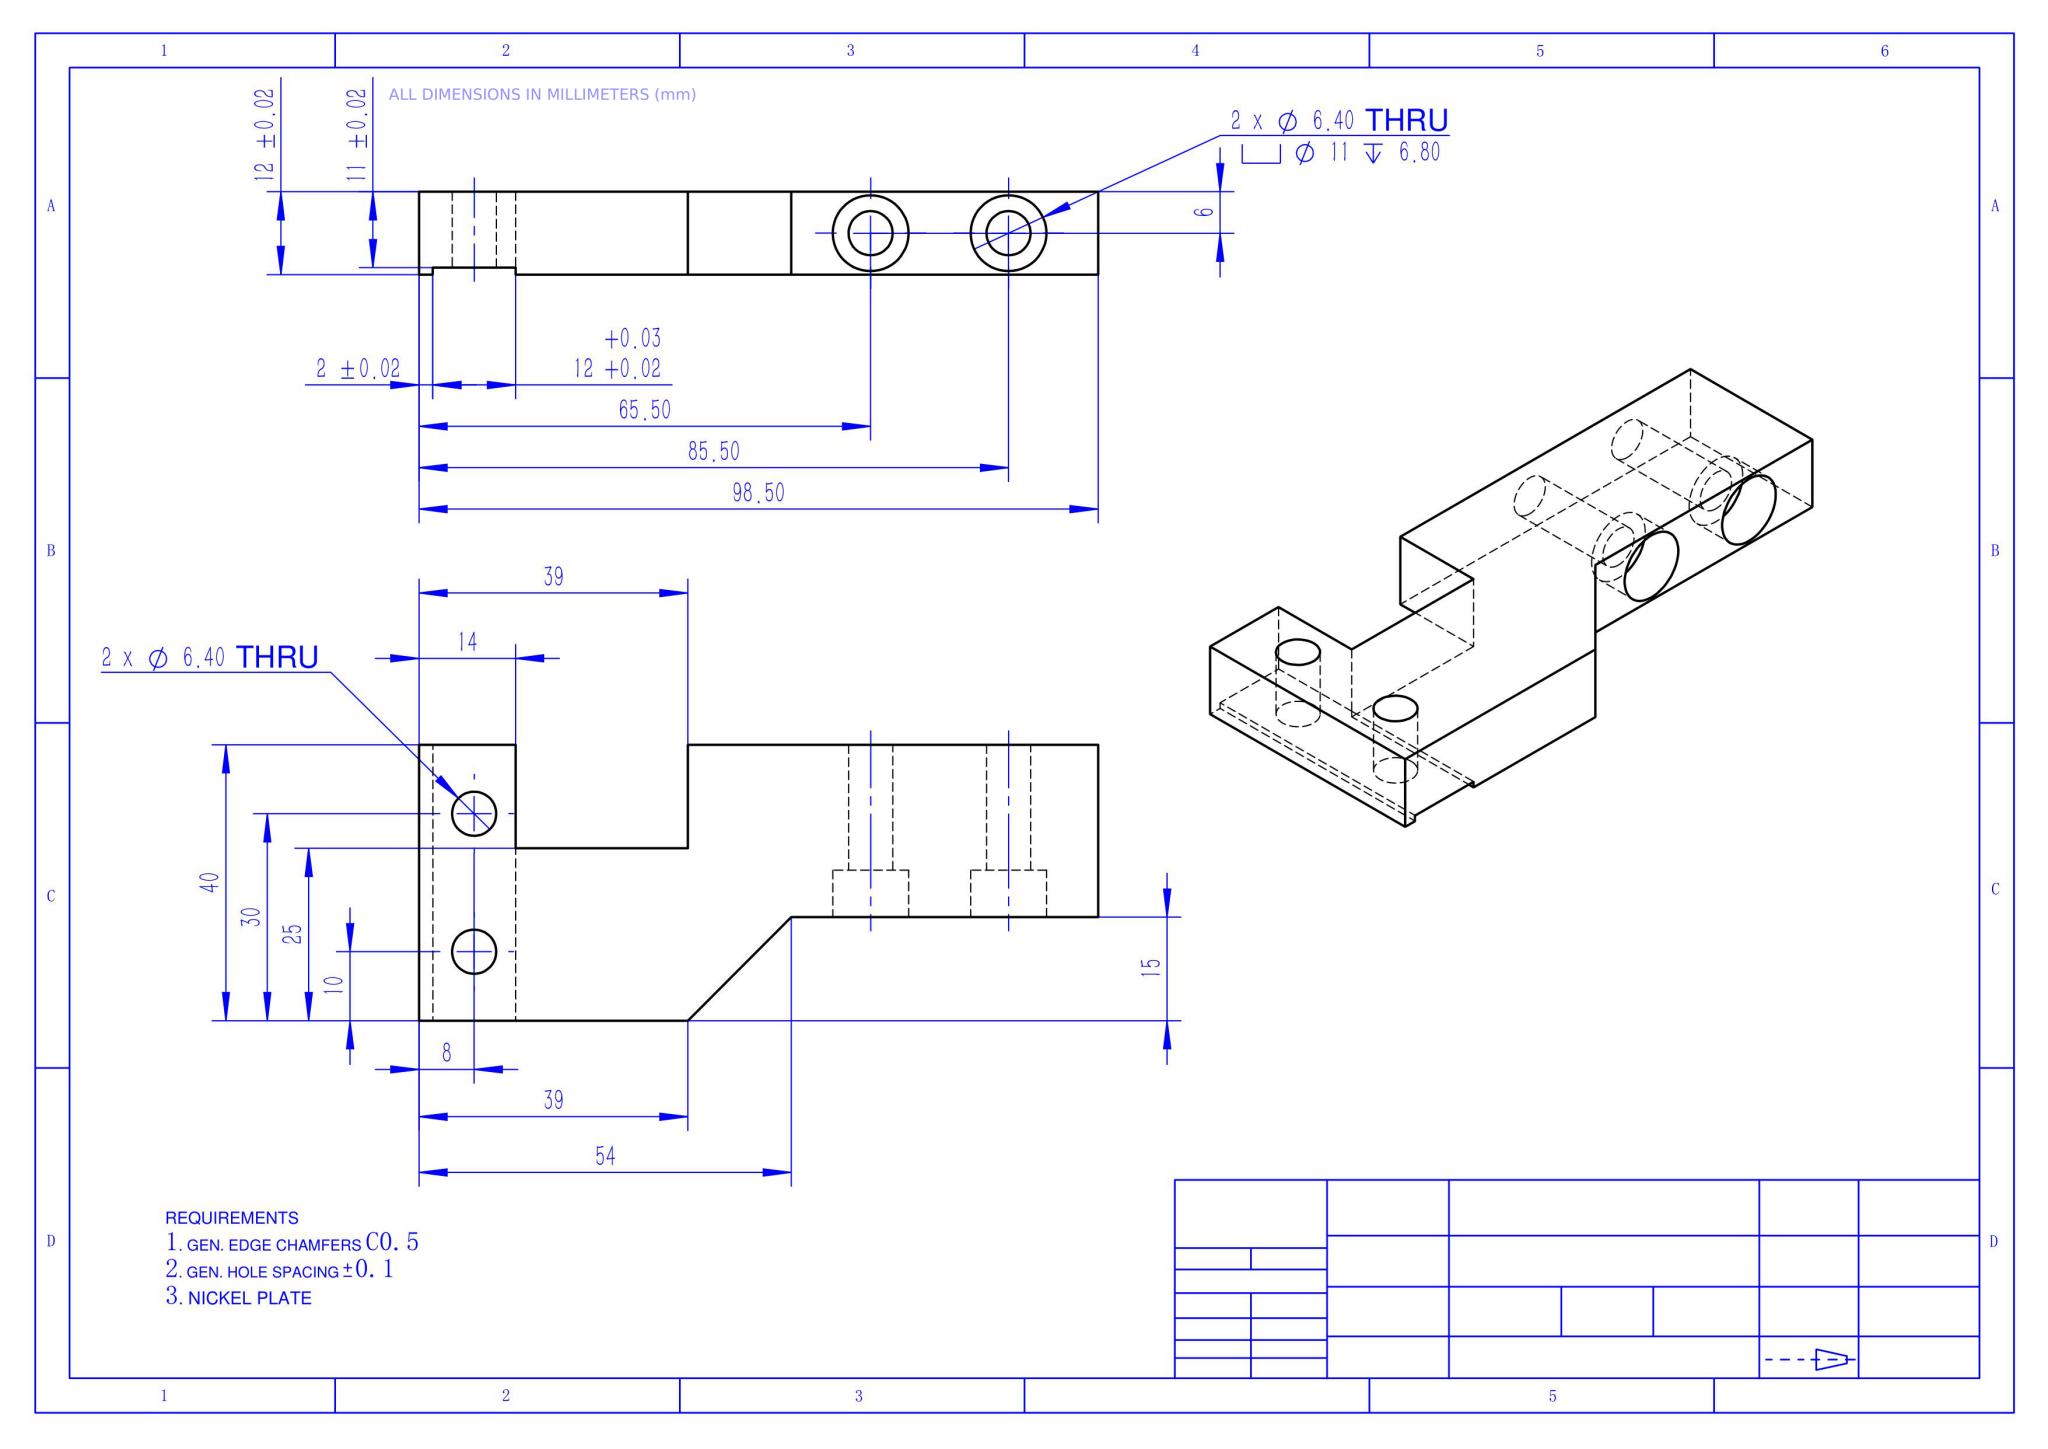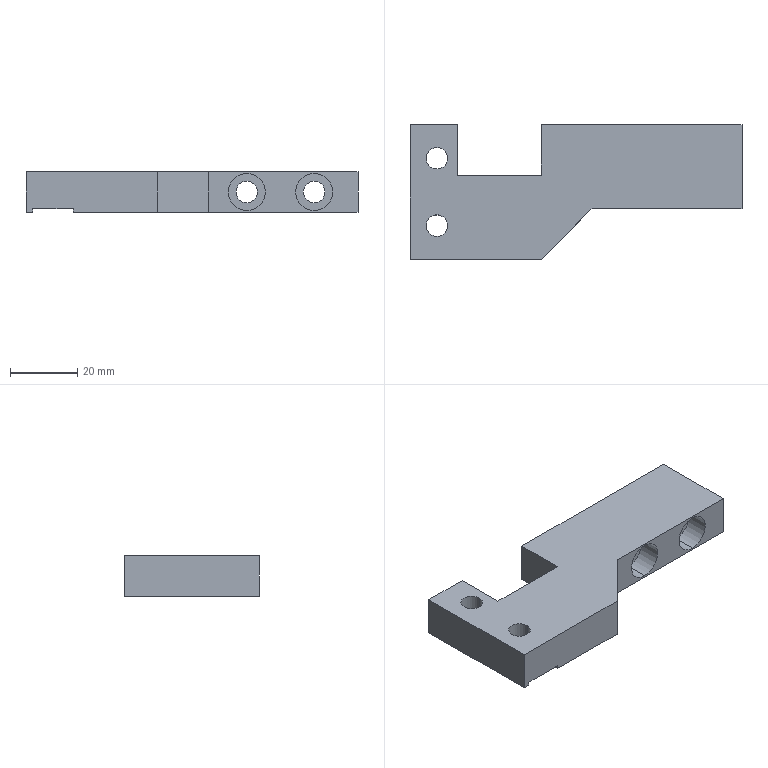Part | NX | mm | 1 solid | 30 faces | box 98.5 x 40 x 12 mm | volume 29769 mm3 | plane 18 | cylinder 12 | commonest cylinder face diameters 6.4 x8 11 x4
STEP:
#1=COLOUR_RGB('',0.698,0.698,0.698);
#2=FILL_AREA_STYLE_COLOUR('',#1);
#3=FILL_AREA_STYLE('',(#2));
#4=SURFACE_STYLE_FILL_AREA(#3);
#5=SURFACE_SIDE_STYLE('',(#4));
#6=SURFACE_STYLE_USAGE(.BOTH.,#5);
#7=PRESENTATION_STYLE_ASSIGNMENT((#6));
#8=CARTESIAN_POINT('',(85.5,1.8,11.5));
#9=VERTEX_POINT('',#8);
#10=CARTESIAN_POINT('',(85.5,1.8,0.5));
#11=VERTEX_POINT('',#10);
#12=CARTESIAN_POINT('',(85.5,1.8,6.));
#13=DIRECTION('',(0.,-1.,0.));
#14=DIRECTION('',(0.,0.,-1.));
#15=AXIS2_PLACEMENT_3D('',#12,#13,#14);
#16=CIRCLE('',#15,5.5);
#17=EDGE_CURVE('',#9,#11,#16,.T.);
#18=ORIENTED_EDGE('',*,*,#17,.F.);
#19=CARTESIAN_POINT('',(85.5,-5.,11.5));
#20=VERTEX_POINT('',#19);
#21=CARTESIAN_POINT('',(85.5,-5.,11.5));
#22=DIRECTION('',(0.,-1.,0.));
#23=VECTOR('',#22,1000.);
#24=LINE('',#21,#23);
#25=EDGE_CURVE('',#9,#20,#24,.T.);
#26=ORIENTED_EDGE('',*,*,#25,.T.);
#27=CARTESIAN_POINT('',(85.5,-5.,0.5));
#28=VERTEX_POINT('',#27);
#29=CARTESIAN_POINT('',(85.5,-5.,6.));
#30=DIRECTION('',(0.,-1.,0.));
#31=DIRECTION('',(0.,0.,-1.));
#32=AXIS2_PLACEMENT_3D('',#29,#30,#31);
#33=CIRCLE('',#32,5.5);
#34=EDGE_CURVE('',#20,#28,#33,.T.);
#35=ORIENTED_EDGE('',*,*,#34,.T.);
#36=CARTESIAN_POINT('',(85.5,-5.,0.5));
#37=DIRECTION('',(0.,-1.,0.));
#38=VECTOR('',#37,1000.);
#39=LINE('',#36,#38);
#40=EDGE_CURVE('',#11,#28,#39,.T.);
#41=ORIENTED_EDGE('',*,*,#40,.F.);
#42=EDGE_LOOP('',(#18,#26,#35,#41));
#43=FACE_OUTER_BOUND('',#42,.T.);
#44=CARTESIAN_POINT('',(85.5,-5.,6.));
#45=DIRECTION('',(0.,-1.,0.));
#46=DIRECTION('',(0.,0.,-1.));
#47=AXIS2_PLACEMENT_3D('',#44,#45,#46);
#48=CYLINDRICAL_SURFACE('',#47,5.5);
#49=ADVANCED_FACE('',(#43),#48,.F.);
#50=CARTESIAN_POINT('',(85.5,20.,9.2));
#51=VERTEX_POINT('',#50);
#52=CARTESIAN_POINT('',(85.5,20.,2.8));
#53=VERTEX_POINT('',#52);
#54=CARTESIAN_POINT('',(85.5,20.,6.));
#55=DIRECTION('',(0.,-1.,0.));
#56=DIRECTION('',(0.,0.,-1.));
#57=AXIS2_PLACEMENT_3D('',#54,#55,#56);
#58=CIRCLE('',#57,3.2);
#59=EDGE_CURVE('',#51,#53,#58,.T.);
#60=ORIENTED_EDGE('',*,*,#59,.F.);
#61=CARTESIAN_POINT('',(85.5,1.8,9.2));
#62=VERTEX_POINT('',#61);
#63=CARTESIAN_POINT('',(85.5,-5.,9.2));
#64=DIRECTION('',(0.,-1.,0.));
#65=VECTOR('',#64,1000.);
#66=LINE('',#63,#65);
#67=EDGE_CURVE('',#51,#62,#66,.T.);
#68=ORIENTED_EDGE('',*,*,#67,.T.);
#69=CARTESIAN_POINT('',(85.5,1.8,2.8));
#70=VERTEX_POINT('',#69);
#71=CARTESIAN_POINT('',(85.5,1.8,6.));
#72=DIRECTION('',(0.,-1.,0.));
#73=DIRECTION('',(0.,0.,-1.));
#74=AXIS2_PLACEMENT_3D('',#71,#72,#73);
#75=CIRCLE('',#74,3.2);
#76=EDGE_CURVE('',#62,#70,#75,.T.);
#77=ORIENTED_EDGE('',*,*,#76,.T.);
#78=CARTESIAN_POINT('',(85.5,-5.,2.8));
#79=DIRECTION('',(0.,-1.,0.));
#80=VECTOR('',#79,1000.);
#81=LINE('',#78,#80);
#82=EDGE_CURVE('',#53,#70,#81,.T.);
#83=ORIENTED_EDGE('',*,*,#82,.F.);
#84=EDGE_LOOP('',(#60,#68,#77,#83));
#85=FACE_OUTER_BOUND('',#84,.T.);
#86=CARTESIAN_POINT('',(85.5,-5.,6.));
#87=DIRECTION('',(0.,-1.,0.));
#88=DIRECTION('',(0.,0.,-1.));
#89=AXIS2_PLACEMENT_3D('',#86,#87,#88);
#90=CYLINDRICAL_SURFACE('',#89,3.2);
#91=ADVANCED_FACE('',(#85),#90,.F.);
#92=CARTESIAN_POINT('',(65.5,1.8,11.5));
#93=VERTEX_POINT('',#92);
#94=CARTESIAN_POINT('',(65.5,1.8,0.5));
#95=VERTEX_POINT('',#94);
#96=CARTESIAN_POINT('',(65.5,1.8,6.));
#97=DIRECTION('',(0.,-1.,0.));
#98=DIRECTION('',(0.,0.,-1.));
#99=AXIS2_PLACEMENT_3D('',#96,#97,#98);
#100=CIRCLE('',#99,5.5);
#101=EDGE_CURVE('',#93,#95,#100,.T.);
#102=ORIENTED_EDGE('',*,*,#101,.F.);
#103=CARTESIAN_POINT('',(65.5,-5.,11.5));
#104=VERTEX_POINT('',#103);
#105=CARTESIAN_POINT('',(65.5,-5.,11.5));
#106=DIRECTION('',(0.,-1.,0.));
#107=VECTOR('',#106,1000.);
#108=LINE('',#105,#107);
#109=EDGE_CURVE('',#93,#104,#108,.T.);
#110=ORIENTED_EDGE('',*,*,#109,.T.);
#111=CARTESIAN_POINT('',(65.5,-5.,0.5));
#112=VERTEX_POINT('',#111);
#113=CARTESIAN_POINT('',(65.5,-5.,6.));
#114=DIRECTION('',(0.,-1.,0.));
#115=DIRECTION('',(0.,0.,-1.));
#116=AXIS2_PLACEMENT_3D('',#113,#114,#115);
#117=CIRCLE('',#116,5.5);
#118=EDGE_CURVE('',#104,#112,#117,.T.);
#119=ORIENTED_EDGE('',*,*,#118,.T.);
#120=CARTESIAN_POINT('',(65.5,-5.,0.5));
#121=DIRECTION('',(0.,-1.,0.));
#122=VECTOR('',#121,1000.);
#123=LINE('',#120,#122);
#124=EDGE_CURVE('',#95,#112,#123,.T.);
#125=ORIENTED_EDGE('',*,*,#124,.F.);
#126=EDGE_LOOP('',(#102,#110,#119,#125));
#127=FACE_OUTER_BOUND('',#126,.T.);
#128=CARTESIAN_POINT('',(65.5,-5.,6.));
#129=DIRECTION('',(0.,-1.,0.));
#130=DIRECTION('',(0.,0.,-1.));
#131=AXIS2_PLACEMENT_3D('',#128,#129,#130);
#132=CYLINDRICAL_SURFACE('',#131,5.5);
#133=ADVANCED_FACE('',(#127),#132,.F.);
#134=CARTESIAN_POINT('',(65.5,20.,9.2));
#135=VERTEX_POINT('',#134);
#136=CARTESIAN_POINT('',(65.5,20.,2.8));
#137=VERTEX_POINT('',#136);
#138=CARTESIAN_POINT('',(65.5,20.,6.));
#139=DIRECTION('',(0.,-1.,0.));
#140=DIRECTION('',(0.,0.,-1.));
#141=AXIS2_PLACEMENT_3D('',#138,#139,#140);
#142=CIRCLE('',#141,3.2);
#143=EDGE_CURVE('',#135,#137,#142,.T.);
#144=ORIENTED_EDGE('',*,*,#143,.F.);
#145=CARTESIAN_POINT('',(65.5,1.8,9.2));
#146=VERTEX_POINT('',#145);
#147=CARTESIAN_POINT('',(65.5,-5.,9.2));
#148=DIRECTION('',(0.,-1.,0.));
#149=VECTOR('',#148,1000.);
#150=LINE('',#147,#149);
#151=EDGE_CURVE('',#135,#146,#150,.T.);
#152=ORIENTED_EDGE('',*,*,#151,.T.);
#153=CARTESIAN_POINT('',(65.5,1.8,2.8));
#154=VERTEX_POINT('',#153);
#155=CARTESIAN_POINT('',(65.5,1.8,6.));
#156=DIRECTION('',(0.,-1.,0.));
#157=DIRECTION('',(0.,0.,-1.));
#158=AXIS2_PLACEMENT_3D('',#155,#156,#157);
#159=CIRCLE('',#158,3.2);
#160=EDGE_CURVE('',#146,#154,#159,.T.);
#161=ORIENTED_EDGE('',*,*,#160,.T.);
#162=CARTESIAN_POINT('',(65.5,-5.,2.8));
#163=DIRECTION('',(0.,-1.,0.));
#164=VECTOR('',#163,1000.);
#165=LINE('',#162,#164);
#166=EDGE_CURVE('',#137,#154,#165,.T.);
#167=ORIENTED_EDGE('',*,*,#166,.F.);
#168=EDGE_LOOP('',(#144,#152,#161,#167));
#169=FACE_OUTER_BOUND('',#168,.T.);
#170=CARTESIAN_POINT('',(65.5,-5.,6.));
#171=DIRECTION('',(0.,-1.,0.));
#172=DIRECTION('',(0.,0.,-1.));
#173=AXIS2_PLACEMENT_3D('',#170,#171,#172);
#174=CYLINDRICAL_SURFACE('',#173,3.2);
#175=ADVANCED_FACE('',(#169),#174,.F.);
#176=CARTESIAN_POINT('',(4.8,10.,1.));
#177=VERTEX_POINT('',#176);
#178=CARTESIAN_POINT('',(11.2,10.,1.));
#179=VERTEX_POINT('',#178);
#180=CARTESIAN_POINT('',(8.,10.,1.));
#181=DIRECTION('',(0.,0.,1.));
#182=DIRECTION('',(1.,0.,0.));
#183=AXIS2_PLACEMENT_3D('',#180,#181,#182);
#184=CIRCLE('',#183,3.2);
#185=EDGE_CURVE('',#177,#179,#184,.T.);
#186=ORIENTED_EDGE('',*,*,#185,.F.);
#187=CARTESIAN_POINT('',(4.8,10.,12.));
#188=VERTEX_POINT('',#187);
#189=CARTESIAN_POINT('',(4.8,10.,12.));
#190=DIRECTION('',(0.,0.,1.));
#191=VECTOR('',#190,1000.);
#192=LINE('',#189,#191);
#193=EDGE_CURVE('',#177,#188,#192,.T.);
#194=ORIENTED_EDGE('',*,*,#193,.T.);
#195=CARTESIAN_POINT('',(11.2,10.,12.));
#196=VERTEX_POINT('',#195);
#197=CARTESIAN_POINT('',(8.,10.,12.));
#198=DIRECTION('',(0.,0.,1.));
#199=DIRECTION('',(1.,0.,0.));
#200=AXIS2_PLACEMENT_3D('',#197,#198,#199);
#201=CIRCLE('',#200,3.2);
#202=EDGE_CURVE('',#188,#196,#201,.T.);
#203=ORIENTED_EDGE('',*,*,#202,.T.);
#204=CARTESIAN_POINT('',(11.2,10.,12.));
#205=DIRECTION('',(0.,0.,1.));
#206=VECTOR('',#205,1000.);
#207=LINE('',#204,#206);
#208=EDGE_CURVE('',#179,#196,#207,.T.);
#209=ORIENTED_EDGE('',*,*,#208,.F.);
#210=EDGE_LOOP('',(#186,#194,#203,#209));
#211=FACE_OUTER_BOUND('',#210,.T.);
#212=CARTESIAN_POINT('',(8.,10.,12.));
#213=DIRECTION('',(0.,0.,1.));
#214=DIRECTION('',(1.,0.,0.));
#215=AXIS2_PLACEMENT_3D('',#212,#213,#214);
#216=CYLINDRICAL_SURFACE('',#215,3.2);
#217=ADVANCED_FACE('',(#211),#216,.F.);
#218=CARTESIAN_POINT('',(4.8,-10.,1.));
#219=VERTEX_POINT('',#218);
#220=CARTESIAN_POINT('',(11.2,-10.,1.));
#221=VERTEX_POINT('',#220);
#222=CARTESIAN_POINT('',(8.,-10.,1.));
#223=DIRECTION('',(0.,0.,1.));
#224=DIRECTION('',(1.,0.,0.));
#225=AXIS2_PLACEMENT_3D('',#222,#223,#224);
#226=CIRCLE('',#225,3.2);
#227=EDGE_CURVE('',#219,#221,#226,.T.);
#228=ORIENTED_EDGE('',*,*,#227,.F.);
#229=CARTESIAN_POINT('',(4.8,-10.,12.));
#230=VERTEX_POINT('',#229);
#231=CARTESIAN_POINT('',(4.8,-10.,12.));
#232=DIRECTION('',(0.,0.,1.));
#233=VECTOR('',#232,1000.);
#234=LINE('',#231,#233);
#235=EDGE_CURVE('',#219,#230,#234,.T.);
#236=ORIENTED_EDGE('',*,*,#235,.T.);
#237=CARTESIAN_POINT('',(11.2,-10.,12.));
#238=VERTEX_POINT('',#237);
#239=CARTESIAN_POINT('',(8.,-10.,12.));
#240=DIRECTION('',(0.,0.,1.));
#241=DIRECTION('',(1.,0.,0.));
#242=AXIS2_PLACEMENT_3D('',#239,#240,#241);
#243=CIRCLE('',#242,3.2);
#244=EDGE_CURVE('',#230,#238,#243,.T.);
#245=ORIENTED_EDGE('',*,*,#244,.T.);
#246=CARTESIAN_POINT('',(11.2,-10.,12.));
#247=DIRECTION('',(0.,0.,1.));
#248=VECTOR('',#247,1000.);
#249=LINE('',#246,#248);
#250=EDGE_CURVE('',#221,#238,#249,.T.);
#251=ORIENTED_EDGE('',*,*,#250,.F.);
#252=EDGE_LOOP('',(#228,#236,#245,#251));
#253=FACE_OUTER_BOUND('',#252,.T.);
#254=CARTESIAN_POINT('',(8.,-10.,12.));
#255=DIRECTION('',(0.,0.,1.));
#256=DIRECTION('',(1.,0.,0.));
#257=AXIS2_PLACEMENT_3D('',#254,#255,#256);
#258=CYLINDRICAL_SURFACE('',#257,3.2);
#259=ADVANCED_FACE('',(#253),#258,.F.);
#260=CARTESIAN_POINT('',(14.,20.,12.));
#261=VERTEX_POINT('',#260);
#262=CARTESIAN_POINT('',(0.,20.,12.));
#263=VERTEX_POINT('',#262);
#264=CARTESIAN_POINT('',(0.,20.,12.));
#265=DIRECTION('',(-1.,0.,0.));
#266=VECTOR('',#265,1000.);
#267=LINE('',#264,#266);
#268=EDGE_CURVE('',#261,#263,#267,.T.);
#269=ORIENTED_EDGE('',*,*,#268,.F.);
#270=CARTESIAN_POINT('',(14.,20.,1.));
#271=VERTEX_POINT('',#270);
#272=CARTESIAN_POINT('',(14.,20.,12.));
#273=DIRECTION('',(0.,0.,-1.));
#274=VECTOR('',#273,1000.);
#275=LINE('',#272,#274);
#276=EDGE_CURVE('',#261,#271,#275,.T.);
#277=ORIENTED_EDGE('',*,*,#276,.T.);
#278=CARTESIAN_POINT('',(2.,20.,1.));
#279=VERTEX_POINT('',#278);
#280=CARTESIAN_POINT('',(2.,20.,1.));
#281=DIRECTION('',(1.,0.,0.));
#282=VECTOR('',#281,1000.);
#283=LINE('',#280,#282);
#284=EDGE_CURVE('',#279,#271,#283,.T.);
#285=ORIENTED_EDGE('',*,*,#284,.F.);
#286=CARTESIAN_POINT('',(2.,20.,0.));
#287=VERTEX_POINT('',#286);
#288=CARTESIAN_POINT('',(2.,20.,1.));
#289=DIRECTION('',(0.,0.,-1.));
#290=VECTOR('',#289,1000.);
#291=LINE('',#288,#290);
#292=EDGE_CURVE('',#279,#287,#291,.T.);
#293=ORIENTED_EDGE('',*,*,#292,.T.);
#294=CARTESIAN_POINT('',(0.,20.,0.));
#295=VERTEX_POINT('',#294);
#296=CARTESIAN_POINT('',(0.,20.,0.));
#297=DIRECTION('',(-1.,0.,0.));
#298=VECTOR('',#297,1000.);
#299=LINE('',#296,#298);
#300=EDGE_CURVE('',#287,#295,#299,.T.);
#301=ORIENTED_EDGE('',*,*,#300,.T.);
#302=CARTESIAN_POINT('',(0.,20.,12.));
#303=DIRECTION('',(0.,0.,-1.));
#304=VECTOR('',#303,1000.);
#305=LINE('',#302,#304);
#306=EDGE_CURVE('',#263,#295,#305,.T.);
#307=ORIENTED_EDGE('',*,*,#306,.F.);
#308=EDGE_LOOP('',(#269,#277,#285,#293,#301,#307));
#309=FACE_OUTER_BOUND('',#308,.T.);
#310=CARTESIAN_POINT('',(0.,20.,12.));
#311=DIRECTION('',(0.,-1.,0.));
#312=DIRECTION('',(0.,0.,-1.));
#313=AXIS2_PLACEMENT_3D('',#310,#311,#312);
#314=PLANE('',#313);
#315=ADVANCED_FACE('',(#309),#314,.F.);
#316=ORIENTED_EDGE('',*,*,#300,.F.);
#317=CARTESIAN_POINT('',(2.,-20.,0.));
#318=VERTEX_POINT('',#317);
#319=CARTESIAN_POINT('',(2.,20.,0.));
#320=DIRECTION('',(0.,1.,0.));
#321=VECTOR('',#320,1000.);
#322=LINE('',#319,#321);
#323=EDGE_CURVE('',#318,#287,#322,.T.);
#324=ORIENTED_EDGE('',*,*,#323,.F.);
#325=CARTESIAN_POINT('',(0.,-20.,0.));
#326=VERTEX_POINT('',#325);
#327=CARTESIAN_POINT('',(0.,-20.,0.));
#328=DIRECTION('',(1.,0.,0.));
#329=VECTOR('',#328,1000.);
#330=LINE('',#327,#329);
#331=EDGE_CURVE('',#326,#318,#330,.T.);
#332=ORIENTED_EDGE('',*,*,#331,.F.);
#333=CARTESIAN_POINT('',(0.,20.,0.));
#334=DIRECTION('',(0.,-1.,0.));
#335=VECTOR('',#334,1000.);
#336=LINE('',#333,#335);
#337=EDGE_CURVE('',#295,#326,#336,.T.);
#338=ORIENTED_EDGE('',*,*,#337,.F.);
#339=EDGE_LOOP('',(#316,#324,#332,#338));
#340=FACE_OUTER_BOUND('',#339,.T.);
#341=CARTESIAN_POINT('',(0.,0.,0.));
#342=DIRECTION('',(0.,0.,1.));
#343=DIRECTION('',(1.,0.,0.));
#344=AXIS2_PLACEMENT_3D('',#341,#342,#343);
#345=PLANE('',#344);
#346=ADVANCED_FACE('',(#340),#345,.F.);
#347=ORIENTED_EDGE('',*,*,#337,.T.);
#348=CARTESIAN_POINT('',(0.,-20.,12.));
#349=VERTEX_POINT('',#348);
#350=CARTESIAN_POINT('',(0.,-20.,12.));
#351=DIRECTION('',(0.,0.,-1.));
#352=VECTOR('',#351,1000.);
#353=LINE('',#350,#352);
#354=EDGE_CURVE('',#349,#326,#353,.T.);
#355=ORIENTED_EDGE('',*,*,#354,.F.);
#356=CARTESIAN_POINT('',(0.,20.,12.));
#357=DIRECTION('',(0.,-1.,0.));
#358=VECTOR('',#357,1000.);
#359=LINE('',#356,#358);
#360=EDGE_CURVE('',#263,#349,#359,.T.);
#361=ORIENTED_EDGE('',*,*,#360,.F.);
#362=ORIENTED_EDGE('',*,*,#306,.T.);
#363=EDGE_LOOP('',(#347,#355,#361,#362));
#364=FACE_OUTER_BOUND('',#363,.T.);
#365=CARTESIAN_POINT('',(0.,20.,12.));
#366=DIRECTION('',(1.,0.,0.));
#367=DIRECTION('',(0.,0.,-1.));
#368=AXIS2_PLACEMENT_3D('',#365,#366,#367);
#369=PLANE('',#368);
#370=ADVANCED_FACE('',(#364),#369,.F.);
#371=CARTESIAN_POINT('',(14.,-20.,0.));
#372=VERTEX_POINT('',#371);
#373=CARTESIAN_POINT('',(39.,-20.,0.));
#374=VERTEX_POINT('',#373);
#375=CARTESIAN_POINT('',(0.,-20.,0.));
#376=DIRECTION('',(1.,0.,0.));
#377=VECTOR('',#376,1000.);
#378=LINE('',#375,#377);
#379=EDGE_CURVE('',#372,#374,#378,.T.);
#380=ORIENTED_EDGE('',*,*,#379,.T.);
#381=CARTESIAN_POINT('',(39.,-20.,12.));
#382=VERTEX_POINT('',#381);
#383=CARTESIAN_POINT('',(39.,-20.,12.));
#384=DIRECTION('',(0.,0.,1.));
#385=VECTOR('',#384,1000.);
#386=LINE('',#383,#385);
#387=EDGE_CURVE('',#374,#382,#386,.T.);
#388=ORIENTED_EDGE('',*,*,#387,.T.);
#389=CARTESIAN_POINT('',(0.,-20.,12.));
#390=DIRECTION('',(1.,0.,0.));
#391=VECTOR('',#390,1000.);
#392=LINE('',#389,#391);
#393=EDGE_CURVE('',#349,#382,#392,.T.);
#394=ORIENTED_EDGE('',*,*,#393,.F.);
#395=ORIENTED_EDGE('',*,*,#354,.T.);
#396=ORIENTED_EDGE('',*,*,#331,.T.);
#397=CARTESIAN_POINT('',(2.,-20.,1.));
#398=VERTEX_POINT('',#397);
#399=CARTESIAN_POINT('',(2.,-20.,1.));
#400=DIRECTION('',(0.,0.,-1.));
#401=VECTOR('',#400,1000.);
#402=LINE('',#399,#401);
#403=EDGE_CURVE('',#398,#318,#402,.T.);
#404=ORIENTED_EDGE('',*,*,#403,.F.);
#405=CARTESIAN_POINT('',(14.,-20.,1.));
#406=VERTEX_POINT('',#405);
#407=CARTESIAN_POINT('',(2.,-20.,1.));
#408=DIRECTION('',(-1.,0.,0.));
#409=VECTOR('',#408,1000.);
#410=LINE('',#407,#409);
#411=EDGE_CURVE('',#406,#398,#410,.T.);
#412=ORIENTED_EDGE('',*,*,#411,.F.);
#413=CARTESIAN_POINT('',(14.,-20.,1.));
#414=DIRECTION('',(0.,0.,-1.));
#415=VECTOR('',#414,1000.);
#416=LINE('',#413,#415);
#417=EDGE_CURVE('',#406,#372,#416,.T.);
#418=ORIENTED_EDGE('',*,*,#417,.T.);
#419=EDGE_LOOP('',(#380,#388,#394,#395,#396,#404,#412,#418));
#420=FACE_OUTER_BOUND('',#419,.T.);
#421=CARTESIAN_POINT('',(0.,-20.,12.));
#422=DIRECTION('',(0.,1.,0.));
#423=DIRECTION('',(0.,0.,1.));
#424=AXIS2_PLACEMENT_3D('',#421,#422,#423);
#425=PLANE('',#424);
#426=ADVANCED_FACE('',(#420),#425,.F.);
#427=CARTESIAN_POINT('',(98.5,-5.,12.));
#428=VERTEX_POINT('',#427);
#429=CARTESIAN_POINT('',(98.5,20.,12.));
#430=VERTEX_POINT('',#429);
#431=CARTESIAN_POINT('',(98.5,20.,12.));
#432=DIRECTION('',(0.,1.,0.));
#433=VECTOR('',#432,1000.);
#434=LINE('',#431,#433);
#435=EDGE_CURVE('',#428,#430,#434,.T.);
#436=ORIENTED_EDGE('',*,*,#435,.F.);
#437=CARTESIAN_POINT('',(98.5,-5.,0.));
#438=VERTEX_POINT('',#437);
#439=CARTESIAN_POINT('',(98.5,-5.,0.));
#440=DIRECTION('',(0.,0.,1.));
#441=VECTOR('',#440,1000.);
#442=LINE('',#439,#441);
#443=EDGE_CURVE('',#438,#428,#442,.T.);
#444=ORIENTED_EDGE('',*,*,#443,.F.);
#445=CARTESIAN_POINT('',(98.5,20.,0.));
#446=VERTEX_POINT('',#445);
#447=CARTESIAN_POINT('',(98.5,20.,0.));
#448=DIRECTION('',(0.,1.,0.));
#449=VECTOR('',#448,1000.);
#450=LINE('',#447,#449);
#451=EDGE_CURVE('',#438,#446,#450,.T.);
#452=ORIENTED_EDGE('',*,*,#451,.T.);
#453=CARTESIAN_POINT('',(98.5,20.,12.));
#454=DIRECTION('',(0.,0.,-1.));
#455=VECTOR('',#454,1000.);
#456=LINE('',#453,#455);
#457=EDGE_CURVE('',#430,#446,#456,.T.);
#458=ORIENTED_EDGE('',*,*,#457,.F.);
#459=EDGE_LOOP('',(#436,#444,#452,#458));
#460=FACE_OUTER_BOUND('',#459,.T.);
#461=CARTESIAN_POINT('',(98.5,20.,12.));
#462=DIRECTION('',(-1.,0.,0.));
#463=DIRECTION('',(0.,0.,1.));
#464=AXIS2_PLACEMENT_3D('',#461,#462,#463);
#465=PLANE('',#464);
#466=ADVANCED_FACE('',(#460),#465,.F.);
#467=CARTESIAN_POINT('',(85.5,20.,6.));
#468=DIRECTION('',(0.,-1.,0.));
#469=DIRECTION('',(0.,0.,-1.));
#470=AXIS2_PLACEMENT_3D('',#467,#468,#469);
#471=CIRCLE('',#470,3.2);
#472=EDGE_CURVE('',#53,#51,#471,.T.);
#473=ORIENTED_EDGE('',*,*,#472,.T.);
#474=ORIENTED_EDGE('',*,*,#59,.T.);
#475=EDGE_LOOP('',(#473,#474));
#476=FACE_BOUND('',#475,.T.);
#477=CARTESIAN_POINT('',(65.5,20.,6.));
#478=DIRECTION('',(0.,-1.,0.));
#479=DIRECTION('',(0.,0.,-1.));
#480=AXIS2_PLACEMENT_3D('',#477,#478,#479);
#481=CIRCLE('',#480,3.2);
#482=EDGE_CURVE('',#137,#135,#481,.T.);
#483=ORIENTED_EDGE('',*,*,#482,.T.);
#484=ORIENTED_EDGE('',*,*,#143,.T.);
#485=EDGE_LOOP('',(#483,#484));
#486=FACE_BOUND('',#485,.T.);
#487=CARTESIAN_POINT('',(39.,20.,0.));
#488=VERTEX_POINT('',#487);
#489=CARTESIAN_POINT('',(0.,20.,0.));
#490=DIRECTION('',(-1.,0.,0.));
#491=VECTOR('',#490,1000.);
#492=LINE('',#489,#491);
#493=EDGE_CURVE('',#446,#488,#492,.T.);
#494=ORIENTED_EDGE('',*,*,#493,.T.);
#495=CARTESIAN_POINT('',(39.,20.,12.));
#496=VERTEX_POINT('',#495);
#497=CARTESIAN_POINT('',(39.,20.,12.));
#498=DIRECTION('',(0.,0.,-1.));
#499=VECTOR('',#498,1000.);
#500=LINE('',#497,#499);
#501=EDGE_CURVE('',#496,#488,#500,.T.);
#502=ORIENTED_EDGE('',*,*,#501,.F.);
#503=CARTESIAN_POINT('',(0.,20.,12.));
#504=DIRECTION('',(-1.,0.,0.));
#505=VECTOR('',#504,1000.);
#506=LINE('',#503,#505);
#507=EDGE_CURVE('',#430,#496,#506,.T.);
#508=ORIENTED_EDGE('',*,*,#507,.F.);
#509=ORIENTED_EDGE('',*,*,#457,.T.);
#510=EDGE_LOOP('',(#494,#502,#508,#509));
#511=FACE_OUTER_BOUND('',#510,.T.);
#512=CARTESIAN_POINT('',(0.,20.,12.));
#513=DIRECTION('',(0.,-1.,0.));
#514=DIRECTION('',(0.,0.,-1.));
#515=AXIS2_PLACEMENT_3D('',#512,#513,#514);
#516=PLANE('',#515);
#517=ADVANCED_FACE('',(#476,#486,#511),#516,.F.);
#518=ORIENTED_EDGE('',*,*,#393,.T.);
#519=CARTESIAN_POINT('',(54.,-5.,12.));
#520=VERTEX_POINT('',#519);
#521=CARTESIAN_POINT('',(29.5,-29.5,12.));
#522=DIRECTION('',(0.7071,0.7071,0.));
#523=VECTOR('',#522,1000.);
#524=LINE('',#521,#523);
#525=EDGE_CURVE('',#382,#520,#524,.T.);
#526=ORIENTED_EDGE('',*,*,#525,.T.);
#527=CARTESIAN_POINT('',(98.5,-5.,12.));
#528=DIRECTION('',(-1.,-0.,0.));
#529=VECTOR('',#528,1000.);
#530=LINE('',#527,#529);
#531=EDGE_CURVE('',#428,#520,#530,.T.);
#532=ORIENTED_EDGE('',*,*,#531,.F.);
#533=ORIENTED_EDGE('',*,*,#435,.T.);
#534=ORIENTED_EDGE('',*,*,#507,.T.);
#535=CARTESIAN_POINT('',(39.,5.,12.));
#536=VERTEX_POINT('',#535);
#537=CARTESIAN_POINT('',(39.,20.,12.));
#538=DIRECTION('',(0.,-1.,0.));
#539=VECTOR('',#538,1000.);
#540=LINE('',#537,#539);
#541=EDGE_CURVE('',#496,#536,#540,.T.);
#542=ORIENTED_EDGE('',*,*,#541,.T.);
#543=CARTESIAN_POINT('',(14.,5.,12.));
#544=VERTEX_POINT('',#543);
#545=CARTESIAN_POINT('',(14.,5.,12.));
#546=DIRECTION('',(-1.,-0.,0.));
#547=VECTOR('',#546,1000.);
#548=LINE('',#545,#547);
#549=EDGE_CURVE('',#536,#544,#548,.T.);
#550=ORIENTED_EDGE('',*,*,#549,.T.);
#551=CARTESIAN_POINT('',(14.,20.,12.));
#552=DIRECTION('',(0.,1.,0.));
#553=VECTOR('',#552,1000.);
#554=LINE('',#551,#553);
#555=EDGE_CURVE('',#544,#261,#554,.T.);
#556=ORIENTED_EDGE('',*,*,#555,.T.);
#557=ORIENTED_EDGE('',*,*,#268,.T.);
#558=ORIENTED_EDGE('',*,*,#360,.T.);
#559=EDGE_LOOP('',(#518,#526,#532,#533,#534,#542,#550,#556,#557,#558));
#560=FACE_OUTER_BOUND('',#559,.T.);
#561=CARTESIAN_POINT('',(8.,10.,12.));
#562=DIRECTION('',(0.,0.,1.));
#563=DIRECTION('',(1.,0.,0.));
#564=AXIS2_PLACEMENT_3D('',#561,#562,#563);
#565=CIRCLE('',#564,3.2);
#566=EDGE_CURVE('',#196,#188,#565,.T.);
#567=ORIENTED_EDGE('',*,*,#566,.F.);
#568=ORIENTED_EDGE('',*,*,#202,.F.);
#569=EDGE_LOOP('',(#567,#568));
#570=FACE_BOUND('',#569,.T.);
#571=CARTESIAN_POINT('',(8.,-10.,12.));
#572=DIRECTION('',(0.,0.,1.));
#573=DIRECTION('',(1.,0.,0.));
#574=AXIS2_PLACEMENT_3D('',#571,#572,#573);
#575=CIRCLE('',#574,3.2);
#576=EDGE_CURVE('',#238,#230,#575,.T.);
#577=ORIENTED_EDGE('',*,*,#576,.F.);
#578=ORIENTED_EDGE('',*,*,#244,.F.);
#579=EDGE_LOOP('',(#577,#578));
#580=FACE_BOUND('',#579,.T.);
#581=CARTESIAN_POINT('',(0.,0.,12.));
#582=DIRECTION('',(0.,0.,1.));
#583=DIRECTION('',(1.,0.,0.));
#584=AXIS2_PLACEMENT_3D('',#581,#582,#583);
#585=PLANE('',#584);
#586=ADVANCED_FACE('',(#560,#570,#580),#585,.T.);
#587=CARTESIAN_POINT('',(54.,-5.,0.));
#588=VERTEX_POINT('',#587);
#589=CARTESIAN_POINT('',(98.5,-5.,0.));
#590=DIRECTION('',(-1.,-0.,0.));
#591=VECTOR('',#590,1000.);
#592=LINE('',#589,#591);
#593=EDGE_CURVE('',#438,#588,#592,.T.);
#594=ORIENTED_EDGE('',*,*,#593,.T.);
#595=CARTESIAN_POINT('',(39.,-20.,0.));
#596=DIRECTION('',(-0.7071,-0.7071,0.));
#597=VECTOR('',#596,1000.);
#598=LINE('',#595,#597);
#599=EDGE_CURVE('',#588,#374,#598,.T.);
#600=ORIENTED_EDGE('',*,*,#599,.T.);
#601=ORIENTED_EDGE('',*,*,#379,.F.);
#602=CARTESIAN_POINT('',(14.,5.,0.));
#603=VERTEX_POINT('',#602);
#604=CARTESIAN_POINT('',(14.,20.,0.));
#605=DIRECTION('',(-0.,-1.,0.));
#606=VECTOR('',#605,1000.);
#607=LINE('',#604,#606);
#608=EDGE_CURVE('',#603,#372,#607,.T.);
#609=ORIENTED_EDGE('',*,*,#608,.F.);
#610=CARTESIAN_POINT('',(39.,5.,0.));
#611=VERTEX_POINT('',#610);
#612=CARTESIAN_POINT('',(14.,5.,0.));
#613=DIRECTION('',(-1.,-0.,0.));
#614=VECTOR('',#613,1000.);
#615=LINE('',#612,#614);
#616=EDGE_CURVE('',#611,#603,#615,.T.);
#617=ORIENTED_EDGE('',*,*,#616,.F.);
#618=CARTESIAN_POINT('',(39.,20.,0.));
#619=DIRECTION('',(0.,-1.,0.));
#620=VECTOR('',#619,1000.);
#621=LINE('',#618,#620);
#622=EDGE_CURVE('',#488,#611,#621,.T.);
#623=ORIENTED_EDGE('',*,*,#622,.F.);
#624=ORIENTED_EDGE('',*,*,#493,.F.);
#625=ORIENTED_EDGE('',*,*,#451,.F.);
#626=EDGE_LOOP('',(#594,#600,#601,#609,#617,#623,#624,#625));
#627=FACE_OUTER_BOUND('',#626,.T.);
#628=CARTESIAN_POINT('',(0.,0.,0.));
#629=DIRECTION('',(0.,0.,1.));
#630=DIRECTION('',(1.,0.,0.));
#631=AXIS2_PLACEMENT_3D('',#628,#629,#630);
#632=PLANE('',#631);
#633=ADVANCED_FACE('',(#627),#632,.F.);
#634=ORIENTED_EDGE('',*,*,#323,.T.);
#635=ORIENTED_EDGE('',*,*,#292,.F.);
#636=CARTESIAN_POINT('',(2.,20.,1.));
#637=DIRECTION('',(0.,1.,0.));
#638=VECTOR('',#637,1000.);
#639=LINE('',#636,#638);
#640=EDGE_CURVE('',#398,#279,#639,.T.);
#641=ORIENTED_EDGE('',*,*,#640,.F.);
#642=ORIENTED_EDGE('',*,*,#403,.T.);
#643=EDGE_LOOP('',(#634,#635,#641,#642));
#644=FACE_OUTER_BOUND('',#643,.T.);
#645=CARTESIAN_POINT('',(2.,20.,1.));
#646=DIRECTION('',(-1.,0.,0.));
#647=DIRECTION('',(-0.,-1.,0.));
#648=AXIS2_PLACEMENT_3D('',#645,#646,#647);
#649=PLANE('',#648);
#650=ADVANCED_FACE('',(#644),#649,.F.);
#651=CARTESIAN_POINT('',(14.,5.,1.));
#652=VERTEX_POINT('',#651);
#653=CARTESIAN_POINT('',(14.,20.,1.));
#654=DIRECTION('',(-0.,-1.,0.));
#655=VECTOR('',#654,1000.);
#656=LINE('',#653,#655);
#657=EDGE_CURVE('',#652,#406,#656,.T.);
#658=ORIENTED_EDGE('',*,*,#657,.F.);
#659=CARTESIAN_POINT('',(14.,5.,12.));
#660=DIRECTION('',(0.,0.,-1.));
#661=VECTOR('',#660,1000.);
#662=LINE('',#659,#661);
#663=EDGE_CURVE('',#652,#603,#662,.T.);
#664=ORIENTED_EDGE('',*,*,#663,.T.);
#665=ORIENTED_EDGE('',*,*,#608,.T.);
#666=ORIENTED_EDGE('',*,*,#417,.F.);
#667=EDGE_LOOP('',(#658,#664,#665,#666));
#668=FACE_OUTER_BOUND('',#667,.T.);
#669=CARTESIAN_POINT('',(14.,20.,1.));
#670=DIRECTION('',(1.,-0.,0.));
#671=DIRECTION('',(0.,1.,0.));
#672=AXIS2_PLACEMENT_3D('',#669,#670,#671);
#673=PLANE('',#672);
#674=ADVANCED_FACE('',(#668),#673,.F.);
#675=CARTESIAN_POINT('',(8.,10.,1.));
#676=DIRECTION('',(0.,0.,1.));
#677=DIRECTION('',(1.,0.,0.));
#678=AXIS2_PLACEMENT_3D('',#675,#676,#677);
#679=CIRCLE('',#678,3.2);
#680=EDGE_CURVE('',#179,#177,#679,.T.);
#681=ORIENTED_EDGE('',*,*,#680,.T.);
#682=ORIENTED_EDGE('',*,*,#185,.T.);
#683=EDGE_LOOP('',(#681,#682));
#684=FACE_BOUND('',#683,.T.);
#685=CARTESIAN_POINT('',(8.,-10.,1.));
#686=DIRECTION('',(0.,0.,1.));
#687=DIRECTION('',(1.,0.,0.));
#688=AXIS2_PLACEMENT_3D('',#685,#686,#687);
#689=CIRCLE('',#688,3.2);
#690=EDGE_CURVE('',#221,#219,#689,.T.);
#691=ORIENTED_EDGE('',*,*,#690,.T.);
#692=ORIENTED_EDGE('',*,*,#227,.T.);
#693=EDGE_LOOP('',(#691,#692));
#694=FACE_BOUND('',#693,.T.);
#695=ORIENTED_EDGE('',*,*,#640,.T.);
#696=ORIENTED_EDGE('',*,*,#284,.T.);
#697=CARTESIAN_POINT('',(14.,20.,1.));
#698=DIRECTION('',(-0.,-1.,0.));
#699=VECTOR('',#698,1000.);
#700=LINE('',#697,#699);
#701=EDGE_CURVE('',#271,#652,#700,.T.);
#702=ORIENTED_EDGE('',*,*,#701,.T.);
#703=ORIENTED_EDGE('',*,*,#657,.T.);
#704=ORIENTED_EDGE('',*,*,#411,.T.);
#705=EDGE_LOOP('',(#695,#696,#702,#703,#704));
#706=FACE_OUTER_BOUND('',#705,.T.);
#707=CARTESIAN_POINT('',(0.,0.,1.));
#708=DIRECTION('',(0.,0.,1.));
#709=DIRECTION('',(1.,0.,0.));
#710=AXIS2_PLACEMENT_3D('',#707,#708,#709);
#711=PLANE('',#710);
#712=ADVANCED_FACE('',(#684,#694,#706),#711,.F.);
#713=ORIENTED_EDGE('',*,*,#235,.F.);
#714=ORIENTED_EDGE('',*,*,#690,.F.);
#715=ORIENTED_EDGE('',*,*,#250,.T.);
#716=ORIENTED_EDGE('',*,*,#576,.T.);
#717=EDGE_LOOP('',(#713,#714,#715,#716));
#718=FACE_OUTER_BOUND('',#717,.T.);
#719=CARTESIAN_POINT('',(8.,-10.,12.));
#720=DIRECTION('',(0.,0.,1.));
#721=DIRECTION('',(1.,0.,0.));
#722=AXIS2_PLACEMENT_3D('',#719,#720,#721);
#723=CYLINDRICAL_SURFACE('',#722,3.2);
#724=ADVANCED_FACE('',(#718),#723,.F.);
#725=ORIENTED_EDGE('',*,*,#193,.F.);
#726=ORIENTED_EDGE('',*,*,#680,.F.);
#727=ORIENTED_EDGE('',*,*,#208,.T.);
#728=ORIENTED_EDGE('',*,*,#566,.T.);
#729=EDGE_LOOP('',(#725,#726,#727,#728));
#730=FACE_OUTER_BOUND('',#729,.T.);
#731=CARTESIAN_POINT('',(8.,10.,12.));
#732=DIRECTION('',(0.,0.,1.));
#733=DIRECTION('',(1.,0.,0.));
#734=AXIS2_PLACEMENT_3D('',#731,#732,#733);
#735=CYLINDRICAL_SURFACE('',#734,3.2);
#736=ADVANCED_FACE('',(#730),#735,.F.);
#737=ORIENTED_EDGE('',*,*,#276,.F.);
#738=ORIENTED_EDGE('',*,*,#555,.F.);
#739=CARTESIAN_POINT('',(14.,5.,12.));
#740=DIRECTION('',(0.,0.,-1.));
#741=VECTOR('',#740,1000.);
#742=LINE('',#739,#741);
#743=EDGE_CURVE('',#544,#652,#742,.T.);
#744=ORIENTED_EDGE('',*,*,#743,.T.);
#745=ORIENTED_EDGE('',*,*,#701,.F.);
#746=EDGE_LOOP('',(#737,#738,#744,#745));
#747=FACE_OUTER_BOUND('',#746,.T.);
#748=CARTESIAN_POINT('',(14.,20.,12.));
#749=DIRECTION('',(-1.,0.,0.));
#750=DIRECTION('',(-0.,-1.,0.));
#751=AXIS2_PLACEMENT_3D('',#748,#749,#750);
#752=PLANE('',#751);
#753=ADVANCED_FACE('',(#747),#752,.F.);
#754=ORIENTED_EDGE('',*,*,#616,.T.);
#755=ORIENTED_EDGE('',*,*,#663,.F.);
#756=ORIENTED_EDGE('',*,*,#743,.F.);
#757=ORIENTED_EDGE('',*,*,#549,.F.);
#758=CARTESIAN_POINT('',(39.,5.,12.));
#759=DIRECTION('',(0.,0.,-1.));
#760=VECTOR('',#759,1000.);
#761=LINE('',#758,#760);
#762=EDGE_CURVE('',#536,#611,#761,.T.);
#763=ORIENTED_EDGE('',*,*,#762,.T.);
#764=EDGE_LOOP('',(#754,#755,#756,#757,#763));
#765=FACE_OUTER_BOUND('',#764,.T.);
#766=CARTESIAN_POINT('',(14.,5.,12.));
#767=DIRECTION('',(0.,-1.,0.));
#768=DIRECTION('',(1.,0.,0.));
#769=AXIS2_PLACEMENT_3D('',#766,#767,#768);
#770=PLANE('',#769);
#771=ADVANCED_FACE('',(#765),#770,.F.);
#772=ORIENTED_EDGE('',*,*,#622,.T.);
#773=ORIENTED_EDGE('',*,*,#762,.F.);
#774=ORIENTED_EDGE('',*,*,#541,.F.);
#775=ORIENTED_EDGE('',*,*,#501,.T.);
#776=EDGE_LOOP('',(#772,#773,#774,#775));
#777=FACE_OUTER_BOUND('',#776,.T.);
#778=CARTESIAN_POINT('',(39.,20.,12.));
#779=DIRECTION('',(1.,0.,0.));
#780=DIRECTION('',(0.,0.,-1.));
#781=AXIS2_PLACEMENT_3D('',#778,#779,#780);
#782=PLANE('',#781);
#783=ADVANCED_FACE('',(#777),#782,.F.);
#784=CARTESIAN_POINT('',(85.5,-5.,6.));
#785=DIRECTION('',(0.,-1.,0.));
#786=DIRECTION('',(0.,0.,-1.));
#787=AXIS2_PLACEMENT_3D('',#784,#785,#786);
#788=CIRCLE('',#787,5.5);
#789=EDGE_CURVE('',#28,#20,#788,.T.);
#790=ORIENTED_EDGE('',*,*,#789,.F.);
#791=ORIENTED_EDGE('',*,*,#34,.F.);
#792=EDGE_LOOP('',(#790,#791));
#793=FACE_BOUND('',#792,.T.);
#794=CARTESIAN_POINT('',(65.5,-5.,6.));
#795=DIRECTION('',(0.,-1.,0.));
#796=DIRECTION('',(0.,0.,-1.));
#797=AXIS2_PLACEMENT_3D('',#794,#795,#796);
#798=CIRCLE('',#797,5.5);
#799=EDGE_CURVE('',#112,#104,#798,.T.);
#800=ORIENTED_EDGE('',*,*,#799,.F.);
#801=ORIENTED_EDGE('',*,*,#118,.F.);
#802=EDGE_LOOP('',(#800,#801));
#803=FACE_BOUND('',#802,.T.);
#804=ORIENTED_EDGE('',*,*,#531,.T.);
#805=CARTESIAN_POINT('',(54.,-5.,0.));
#806=DIRECTION('',(0.,0.,1.));
#807=VECTOR('',#806,1000.);
#808=LINE('',#805,#807);
#809=EDGE_CURVE('',#588,#520,#808,.T.);
#810=ORIENTED_EDGE('',*,*,#809,.F.);
#811=ORIENTED_EDGE('',*,*,#593,.F.);
#812=ORIENTED_EDGE('',*,*,#443,.T.);
#813=EDGE_LOOP('',(#804,#810,#811,#812));
#814=FACE_OUTER_BOUND('',#813,.T.);
#815=CARTESIAN_POINT('',(98.5,-5.,0.));
#816=DIRECTION('',(-0.,1.,0.));
#817=DIRECTION('',(-1.,-0.,0.));
#818=AXIS2_PLACEMENT_3D('',#815,#816,#817);
#819=PLANE('',#818);
#820=ADVANCED_FACE('',(#793,#803,#814),#819,.F.);
#821=ORIENTED_EDGE('',*,*,#151,.F.);
#822=ORIENTED_EDGE('',*,*,#482,.F.);
#823=ORIENTED_EDGE('',*,*,#166,.T.);
#824=CARTESIAN_POINT('',(65.5,1.8,6.));
#825=DIRECTION('',(0.,-1.,0.));
#826=DIRECTION('',(0.,0.,-1.));
#827=AXIS2_PLACEMENT_3D('',#824,#825,#826);
#828=CIRCLE('',#827,3.2);
#829=EDGE_CURVE('',#154,#146,#828,.T.);
#830=ORIENTED_EDGE('',*,*,#829,.T.);
#831=EDGE_LOOP('',(#821,#822,#823,#830));
#832=FACE_OUTER_BOUND('',#831,.T.);
#833=CARTESIAN_POINT('',(65.5,-5.,6.));
#834=DIRECTION('',(0.,-1.,0.));
#835=DIRECTION('',(0.,0.,-1.));
#836=AXIS2_PLACEMENT_3D('',#833,#834,#835);
#837=CYLINDRICAL_SURFACE('',#836,3.2);
#838=ADVANCED_FACE('',(#832),#837,.F.);
#839=ORIENTED_EDGE('',*,*,#829,.F.);
#840=ORIENTED_EDGE('',*,*,#160,.F.);
#841=EDGE_LOOP('',(#839,#840));
#842=FACE_BOUND('',#841,.T.);
#843=CARTESIAN_POINT('',(65.5,1.8,6.));
#844=DIRECTION('',(0.,-1.,0.));
#845=DIRECTION('',(0.,0.,-1.));
#846=AXIS2_PLACEMENT_3D('',#843,#844,#845);
#847=CIRCLE('',#846,5.5);
#848=EDGE_CURVE('',#95,#93,#847,.T.);
#849=ORIENTED_EDGE('',*,*,#848,.T.);
#850=ORIENTED_EDGE('',*,*,#101,.T.);
#851=EDGE_LOOP('',(#849,#850));
#852=FACE_OUTER_BOUND('',#851,.T.);
#853=CARTESIAN_POINT('',(68.7,1.8,6.));
#854=DIRECTION('',(0.,1.,0.));
#855=DIRECTION('',(0.,0.,1.));
#856=AXIS2_PLACEMENT_3D('',#853,#854,#855);
#857=PLANE('',#856);
#858=ADVANCED_FACE('',(#842,#852),#857,.F.);
#859=ORIENTED_EDGE('',*,*,#109,.F.);
#860=ORIENTED_EDGE('',*,*,#848,.F.);
#861=ORIENTED_EDGE('',*,*,#124,.T.);
#862=ORIENTED_EDGE('',*,*,#799,.T.);
#863=EDGE_LOOP('',(#859,#860,#861,#862));
#864=FACE_OUTER_BOUND('',#863,.T.);
#865=CARTESIAN_POINT('',(65.5,-5.,6.));
#866=DIRECTION('',(0.,-1.,0.));
#867=DIRECTION('',(0.,0.,-1.));
#868=AXIS2_PLACEMENT_3D('',#865,#866,#867);
#869=CYLINDRICAL_SURFACE('',#868,5.5);
#870=ADVANCED_FACE('',(#864),#869,.F.);
#871=ORIENTED_EDGE('',*,*,#67,.F.);
#872=ORIENTED_EDGE('',*,*,#472,.F.);
#873=ORIENTED_EDGE('',*,*,#82,.T.);
#874=CARTESIAN_POINT('',(85.5,1.8,6.));
#875=DIRECTION('',(0.,-1.,0.));
#876=DIRECTION('',(0.,0.,-1.));
#877=AXIS2_PLACEMENT_3D('',#874,#875,#876);
#878=CIRCLE('',#877,3.2);
#879=EDGE_CURVE('',#70,#62,#878,.T.);
#880=ORIENTED_EDGE('',*,*,#879,.T.);
#881=EDGE_LOOP('',(#871,#872,#873,#880));
#882=FACE_OUTER_BOUND('',#881,.T.);
#883=CARTESIAN_POINT('',(85.5,-5.,6.));
#884=DIRECTION('',(0.,-1.,0.));
#885=DIRECTION('',(0.,0.,-1.));
#886=AXIS2_PLACEMENT_3D('',#883,#884,#885);
#887=CYLINDRICAL_SURFACE('',#886,3.2);
#888=ADVANCED_FACE('',(#882),#887,.F.);
#889=ORIENTED_EDGE('',*,*,#879,.F.);
#890=ORIENTED_EDGE('',*,*,#76,.F.);
#891=EDGE_LOOP('',(#889,#890));
#892=FACE_BOUND('',#891,.T.);
#893=CARTESIAN_POINT('',(85.5,1.8,6.));
#894=DIRECTION('',(0.,-1.,0.));
#895=DIRECTION('',(0.,0.,-1.));
#896=AXIS2_PLACEMENT_3D('',#893,#894,#895);
#897=CIRCLE('',#896,5.5);
#898=EDGE_CURVE('',#11,#9,#897,.T.);
#899=ORIENTED_EDGE('',*,*,#898,.T.);
#900=ORIENTED_EDGE('',*,*,#17,.T.);
#901=EDGE_LOOP('',(#899,#900));
#902=FACE_OUTER_BOUND('',#901,.T.);
#903=CARTESIAN_POINT('',(88.7,1.8,6.));
#904=DIRECTION('',(0.,1.,0.));
#905=DIRECTION('',(0.,0.,1.));
#906=AXIS2_PLACEMENT_3D('',#903,#904,#905);
#907=PLANE('',#906);
#908=ADVANCED_FACE('',(#892,#902),#907,.F.);
#909=ORIENTED_EDGE('',*,*,#25,.F.);
#910=ORIENTED_EDGE('',*,*,#898,.F.);
#911=ORIENTED_EDGE('',*,*,#40,.T.);
#912=ORIENTED_EDGE('',*,*,#789,.T.);
#913=EDGE_LOOP('',(#909,#910,#911,#912));
#914=FACE_OUTER_BOUND('',#913,.T.);
#915=CARTESIAN_POINT('',(85.5,-5.,6.));
#916=DIRECTION('',(0.,-1.,0.));
#917=DIRECTION('',(0.,0.,-1.));
#918=AXIS2_PLACEMENT_3D('',#915,#916,#917);
#919=CYLINDRICAL_SURFACE('',#918,5.5);
#920=ADVANCED_FACE('',(#914),#919,.F.);
#921=ORIENTED_EDGE('',*,*,#599,.F.);
#922=ORIENTED_EDGE('',*,*,#809,.T.);
#923=ORIENTED_EDGE('',*,*,#525,.F.);
#924=ORIENTED_EDGE('',*,*,#387,.F.);
#925=EDGE_LOOP('',(#921,#922,#923,#924));
#926=FACE_OUTER_BOUND('',#925,.T.);
#927=CARTESIAN_POINT('',(39.,-20.,12.));
#928=DIRECTION('',(-0.7071,0.7071,0.));
#929=DIRECTION('',(0.,0.,1.));
#930=AXIS2_PLACEMENT_3D('',#927,#928,#929);
#931=PLANE('',#930);
#932=ADVANCED_FACE('',(#926),#931,.F.);
#933=CLOSED_SHELL('',(#49,#91,#133,#175,#217,#259,#315,#346,#370,#426,#466,#517,#586,#633,#650,#674,#712,#724,#736,#753,#771,#783,#820,#838,#858,#870,#888,#908,#920,#932));
#934=MANIFOLD_SOLID_BREP('',#933);
#935=CARTESIAN_POINT('',(0.,0.,0.));
#936=DIRECTION('',(0.,0.,1.));
#937=DIRECTION('',(1.,0.,0.));
#938=AXIS2_PLACEMENT_3D('',#935,#936,#937);
#939=(LENGTH_UNIT()NAMED_UNIT(*)SI_UNIT(.MILLI.,.METRE.));
#940=UNCERTAINTY_MEASURE_WITH_UNIT(LENGTH_MEASURE(0.00001),#939,'','');
#941=(NAMED_UNIT(*)PLANE_ANGLE_UNIT()SI_UNIT($,.RADIAN.));
#942=(NAMED_UNIT(*)SI_UNIT($,.STERADIAN.)SOLID_ANGLE_UNIT());
#943=(GEOMETRIC_REPRESENTATION_CONTEXT(3)GLOBAL_UNCERTAINTY_ASSIGNED_CONTEXT((#940))GLOBAL_UNIT_ASSIGNED_CONTEXT((#939,#941,#942))REPRESENTATION_CONTEXT('',''));
#944=ADVANCED_BREP_SHAPE_REPRESENTATION('',(#934,#938),#943);
#945=STYLED_ITEM('',(#7),#944);
#946=PRESENTATION_LAYER_ASSIGNMENT('','',(#945));
#947=COLOUR_RGB('',0.698,0.698,0.698);
#948=FILL_AREA_STYLE_COLOUR('',#947);
#949=FILL_AREA_STYLE('',(#948));
#950=SURFACE_STYLE_FILL_AREA(#949);
#951=SURFACE_SIDE_STYLE('',(#950));
#952=SURFACE_STYLE_USAGE(.BOTH.,#951);
#953=PRESENTATION_STYLE_ASSIGNMENT((#952));
#954=STYLED_ITEM('',(#953),#934);
#955=PRESENTATION_LAYER_ASSIGNMENT('','',(#954));
#956=(LENGTH_UNIT()NAMED_UNIT(*)SI_UNIT(.MILLI.,.METRE.));
#957=UNCERTAINTY_MEASURE_WITH_UNIT(LENGTH_MEASURE(0.00001),#956,'','');
#958=(NAMED_UNIT(*)PLANE_ANGLE_UNIT()SI_UNIT($,.RADIAN.));
#959=(NAMED_UNIT(*)SI_UNIT($,.STERADIAN.)SOLID_ANGLE_UNIT());
#960=(GEOMETRIC_REPRESENTATION_CONTEXT(3)GLOBAL_UNCERTAINTY_ASSIGNED_CONTEXT((#957))GLOBAL_UNIT_ASSIGNED_CONTEXT((#956,#958,#959))REPRESENTATION_CONTEXT('',''));
#961=MECHANICAL_DESIGN_GEOMETRIC_PRESENTATION_REPRESENTATION('',(#945),#960);
#962=(LENGTH_UNIT()NAMED_UNIT(*)SI_UNIT(.MILLI.,.METRE.));
#963=UNCERTAINTY_MEASURE_WITH_UNIT(LENGTH_MEASURE(0.00001),#962,'','');
#964=(NAMED_UNIT(*)PLANE_ANGLE_UNIT()SI_UNIT($,.RADIAN.));
#965=(NAMED_UNIT(*)SI_UNIT($,.STERADIAN.)SOLID_ANGLE_UNIT());
#966=(GEOMETRIC_REPRESENTATION_CONTEXT(3)GLOBAL_UNCERTAINTY_ASSIGNED_CONTEXT((#963))GLOBAL_UNIT_ASSIGNED_CONTEXT((#962,#964,#965))REPRESENTATION_CONTEXT('',''));
#967=MECHANICAL_DESIGN_GEOMETRIC_PRESENTATION_REPRESENTATION('',(#954),#966);